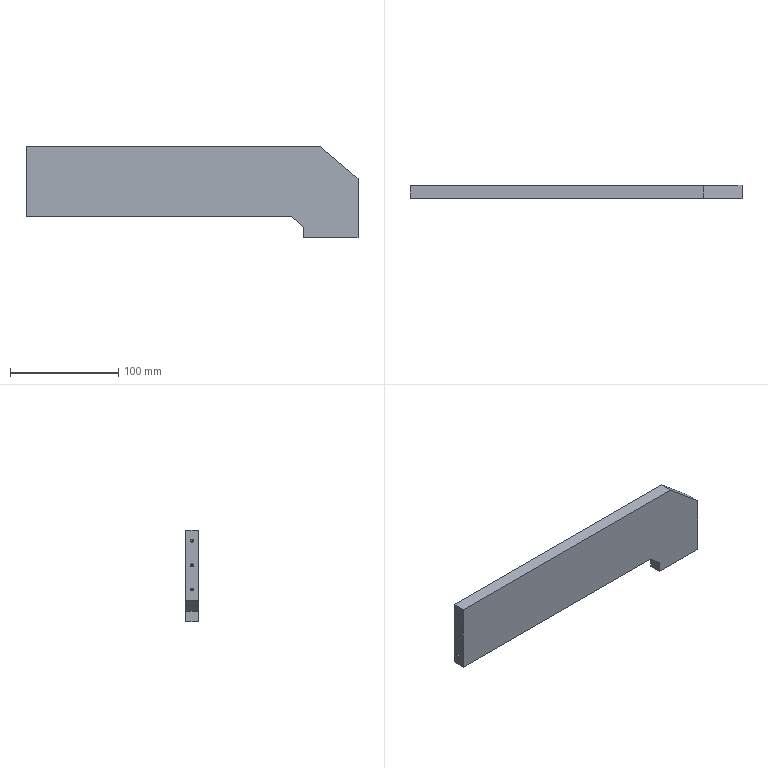Component | SolidWorks | RobotArmCrossPlate1-1 | 1 solid | 34 faces | box 307 x 12 x 85 mm | volume 244874 mm3 | cylinder 12 | cone 12 | plane 10 | commonest cylinder face diameters 4.2 x6 2.5 x6
build123d program:
from build123d import *

# Parameters (mm, degrees)
SKETCH1_W                 = 65
SKETCH1_H                 = 307
BOSS_EXTRUDE1_DEPTH       = 12
SKETCH2_W                 = 85
SKETCH2_H                 = 50
BOSS_EXTRUDE2_DEPTH       = 12
CHAMFER2_SIZE             = 30
CHAMFER2_SIZE2            = 35.753
CHAMFER3_SIZE             = 10
CHAMFER3_SIZE2            = 11.918
M3X0_5_TAPPED_HOLE1_D     = 2.5
M3X0_5_TAPPED_HOLE1_DEPTH = 15
M3X0_5_TAPPED_HOLE1_TIP   = 0.7511
M5X0_8_TAPPED_HOLE1_D     = 4.2
M5X0_8_TAPPED_HOLE1_DEPTH = 15
M5X0_8_TAPPED_HOLE1_TIP   = 1.262


with BuildPart() as part:
    # Sketch1 → Boss-Extrude1 (new body)
    with BuildSketch(Plane.XY):
        Rectangle(SKETCH1_W, SKETCH1_H)
    extrude(amount=BOSS_EXTRUDE1_DEPTH)

    # Sketch2 → Boss-Extrude2 (add)
    with BuildSketch(Plane.XY.offset(12)):
        with Locations((10, 128.5)):
            Rectangle(SKETCH2_W, SKETCH2_H)
    extrude(amount=-BOSS_EXTRUDE2_DEPTH)

    # Chamfer2
    chamfer2_edges = [part.edges().sort_by_distance(p)[0] for p in [
        (-32.5, 153.5, 6),
    ]]
    chamfer2_side = [part.faces().sort_by_distance(p)[0] for p in [
        (10, 153.5, 6),
    ]]
    chamfer(chamfer2_edges, length=CHAMFER2_SIZE, length2=CHAMFER2_SIZE2, reference=chamfer2_side[0])

    # Chamfer3
    chamfer3_edges = [part.edges().sort_by_distance(p)[0] for p in [
        (32.5, 103.5, 6),
    ]]
    chamfer3_side = [part.faces().sort_by_distance(p)[0] for p in [
        (42.5, 103.5, 6),
    ]]
    chamfer(chamfer3_edges, length=CHAMFER3_SIZE, length2=CHAMFER3_SIZE2, reference=chamfer3_side[0])

    # M3x0.5 Tapped Hole1
    with Locations(Plane(origin=(0, -153.5, 0), x_dir=(-1, 0, 0), z_dir=(0, -1, 0))):
        with Locations((22.5, -6), (0, -6), (-22.5, -6)):
            Hole(M3X0_5_TAPPED_HOLE1_D / 2, depth=M3X0_5_TAPPED_HOLE1_DEPTH)
            with Locations((0, 0, -(M3X0_5_TAPPED_HOLE1_DEPTH + M3X0_5_TAPPED_HOLE1_TIP / 2))):  # 118° drill point
                Cone(0, M3X0_5_TAPPED_HOLE1_D / 2, M3X0_5_TAPPED_HOLE1_TIP, mode=Mode.SUBTRACT)

    # M5x0.8 Tapped Hole1
    with Locations(Plane(origin=(52.5, 0, 0), x_dir=(0, 0, -1), z_dir=(1, 0, 0))):
        with Locations((-6, 148.5), (-6, 128.5), (-6.289, 108.5)):
            Hole(M5X0_8_TAPPED_HOLE1_D / 2, depth=M5X0_8_TAPPED_HOLE1_DEPTH)
            with Locations((0, 0, -(M5X0_8_TAPPED_HOLE1_DEPTH + M5X0_8_TAPPED_HOLE1_TIP / 2))):  # 118° drill point
                Cone(0, M5X0_8_TAPPED_HOLE1_D / 2, M5X0_8_TAPPED_HOLE1_TIP, mode=Mode.SUBTRACT)


solid = part.part

# Placed as in the assembly
solid = solid.moved(Location((-174.022, 67.945, 113.051), (90, 0, -90)))
STEP:
#1=COLOUR_RGB('',0.7922,0.8196,0.9333);
#2=FILL_AREA_STYLE_COLOUR('',#1);
#3=FILL_AREA_STYLE('',(#2));
#4=SURFACE_STYLE_FILL_AREA(#3);
#5=SURFACE_SIDE_STYLE('',(#4));
#6=SURFACE_STYLE_USAGE(.BOTH.,#5);
#7=PRESENTATION_STYLE_ASSIGNMENT((#6));
#8=CARTESIAN_POINT('',(-1.005,2.356,2.974));
#9=VERTEX_POINT('',#8);
#10=CARTESIAN_POINT('',(-1.005,2.521,2.974));
#11=VERTEX_POINT('',#10);
#12=CARTESIAN_POINT('',(-1.005,2.439,2.974));
#13=DIRECTION('',(-0.,0.,-1.));
#14=DIRECTION('',(0.,1.,0.));
#15=AXIS2_PLACEMENT_3D('',#12,#13,#14);
#16=CIRCLE('',#15,0.08268);
#17=EDGE_CURVE('',#9,#11,#16,.T.);
#18=ORIENTED_EDGE('',*,*,#17,.F.);
#19=CARTESIAN_POINT('',(-1.005,2.356,2.384));
#20=VERTEX_POINT('',#19);
#21=CARTESIAN_POINT('',(-1.005,2.356,2.384));
#22=DIRECTION('',(-0.,0.,-1.));
#23=VECTOR('',#22,39.37);
#24=LINE('',#21,#23);
#25=EDGE_CURVE('',#9,#20,#24,.T.);
#26=ORIENTED_EDGE('',*,*,#25,.T.);
#27=CARTESIAN_POINT('',(-1.005,2.521,2.384));
#28=VERTEX_POINT('',#27);
#29=CARTESIAN_POINT('',(-1.005,2.439,2.384));
#30=DIRECTION('',(-0.,0.,-1.));
#31=DIRECTION('',(0.,1.,0.));
#32=AXIS2_PLACEMENT_3D('',#29,#30,#31);
#33=CIRCLE('',#32,0.08268);
#34=EDGE_CURVE('',#20,#28,#33,.T.);
#35=ORIENTED_EDGE('',*,*,#34,.T.);
#36=CARTESIAN_POINT('',(-1.005,2.521,2.384));
#37=DIRECTION('',(-0.,0.,-1.));
#38=VECTOR('',#37,39.37);
#39=LINE('',#36,#38);
#40=EDGE_CURVE('',#11,#28,#39,.T.);
#41=ORIENTED_EDGE('',*,*,#40,.F.);
#42=EDGE_LOOP('',(#18,#26,#35,#41));
#43=FACE_OUTER_BOUND('',#42,.T.);
#44=CARTESIAN_POINT('',(-1.005,2.439,2.384));
#45=DIRECTION('',(-0.,0.,-1.));
#46=DIRECTION('',(0.,1.,0.));
#47=AXIS2_PLACEMENT_3D('',#44,#45,#46);
#48=CYLINDRICAL_SURFACE('',#47,0.08268);
#49=ADVANCED_FACE('',(#43),#48,.F.);
#50=CARTESIAN_POINT('',(-1.005,2.439,3.024));
#51=VERTEX_POINT('',#50);
#52=CARTESIAN_POINT('',(-1.005,2.521,2.974));
#53=DIRECTION('',(-0.,0.8572,-0.515));
#54=VECTOR('',#53,39.37);
#55=LINE('',#52,#54);
#56=EDGE_CURVE('',#51,#11,#55,.T.);
#57=ORIENTED_EDGE('',*,*,#56,.F.);
#58=CARTESIAN_POINT('',(-1.005,2.356,2.974));
#59=DIRECTION('',(0.,-0.8572,-0.515));
#60=VECTOR('',#59,39.37);
#61=LINE('',#58,#60);
#62=EDGE_CURVE('',#51,#9,#61,.T.);
#63=ORIENTED_EDGE('',*,*,#62,.T.);
#64=ORIENTED_EDGE('',*,*,#17,.T.);
#65=EDGE_LOOP('',(#57,#63,#64));
#66=FACE_OUTER_BOUND('',#65,.T.);
#67=CARTESIAN_POINT('',(-1.005,2.439,2.974));
#68=DIRECTION('',(-0.,0.,-1.));
#69=DIRECTION('',(0.,1.,0.));
#70=AXIS2_PLACEMENT_3D('',#67,#68,#69);
#71=CONICAL_SURFACE('',#70,0.08268,1.03);
#72=ADVANCED_FACE('',(#66),#71,.F.);
#73=CARTESIAN_POINT('',(-1.792,2.356,2.974));
#74=VERTEX_POINT('',#73);
#75=CARTESIAN_POINT('',(-1.792,2.521,2.974));
#76=VERTEX_POINT('',#75);
#77=CARTESIAN_POINT('',(-1.792,2.439,2.974));
#78=DIRECTION('',(-0.,0.,-1.));
#79=DIRECTION('',(0.,1.,0.));
#80=AXIS2_PLACEMENT_3D('',#77,#78,#79);
#81=CIRCLE('',#80,0.08268);
#82=EDGE_CURVE('',#74,#76,#81,.T.);
#83=ORIENTED_EDGE('',*,*,#82,.F.);
#84=CARTESIAN_POINT('',(-1.792,2.356,2.384));
#85=VERTEX_POINT('',#84);
#86=CARTESIAN_POINT('',(-1.792,2.356,2.384));
#87=DIRECTION('',(-0.,0.,-1.));
#88=VECTOR('',#87,39.37);
#89=LINE('',#86,#88);
#90=EDGE_CURVE('',#74,#85,#89,.T.);
#91=ORIENTED_EDGE('',*,*,#90,.T.);
#92=CARTESIAN_POINT('',(-1.792,2.521,2.384));
#93=VERTEX_POINT('',#92);
#94=CARTESIAN_POINT('',(-1.792,2.439,2.384));
#95=DIRECTION('',(-0.,0.,-1.));
#96=DIRECTION('',(0.,1.,0.));
#97=AXIS2_PLACEMENT_3D('',#94,#95,#96);
#98=CIRCLE('',#97,0.08268);
#99=EDGE_CURVE('',#85,#93,#98,.T.);
#100=ORIENTED_EDGE('',*,*,#99,.T.);
#101=CARTESIAN_POINT('',(-1.792,2.521,2.384));
#102=DIRECTION('',(-0.,0.,-1.));
#103=VECTOR('',#102,39.37);
#104=LINE('',#101,#103);
#105=EDGE_CURVE('',#76,#93,#104,.T.);
#106=ORIENTED_EDGE('',*,*,#105,.F.);
#107=EDGE_LOOP('',(#83,#91,#100,#106));
#108=FACE_OUTER_BOUND('',#107,.T.);
#109=CARTESIAN_POINT('',(-1.792,2.439,2.384));
#110=DIRECTION('',(-0.,0.,-1.));
#111=DIRECTION('',(0.,1.,0.));
#112=AXIS2_PLACEMENT_3D('',#109,#110,#111);
#113=CYLINDRICAL_SURFACE('',#112,0.08268);
#114=ADVANCED_FACE('',(#108),#113,.F.);
#115=CARTESIAN_POINT('',(-1.792,2.439,3.024));
#116=VERTEX_POINT('',#115);
#117=CARTESIAN_POINT('',(-1.792,2.521,2.974));
#118=DIRECTION('',(-0.,0.8572,-0.515));
#119=VECTOR('',#118,39.37);
#120=LINE('',#117,#119);
#121=EDGE_CURVE('',#116,#76,#120,.T.);
#122=ORIENTED_EDGE('',*,*,#121,.F.);
#123=CARTESIAN_POINT('',(-1.792,2.356,2.974));
#124=DIRECTION('',(0.,-0.8572,-0.515));
#125=VECTOR('',#124,39.37);
#126=LINE('',#123,#125);
#127=EDGE_CURVE('',#116,#74,#126,.T.);
#128=ORIENTED_EDGE('',*,*,#127,.T.);
#129=ORIENTED_EDGE('',*,*,#82,.T.);
#130=EDGE_LOOP('',(#122,#128,#129));
#131=FACE_OUTER_BOUND('',#130,.T.);
#132=CARTESIAN_POINT('',(-1.792,2.439,2.974));
#133=DIRECTION('',(-0.,0.,-1.));
#134=DIRECTION('',(0.,1.,0.));
#135=AXIS2_PLACEMENT_3D('',#132,#133,#134);
#136=CONICAL_SURFACE('',#135,0.08268,1.03);
#137=ADVANCED_FACE('',(#131),#136,.F.);
#138=CARTESIAN_POINT('',(-2.58,2.345,2.974));
#139=VERTEX_POINT('',#138);
#140=CARTESIAN_POINT('',(-2.58,2.51,2.974));
#141=VERTEX_POINT('',#140);
#142=CARTESIAN_POINT('',(-2.58,2.427,2.974));
#143=DIRECTION('',(-0.,0.,-1.));
#144=DIRECTION('',(0.,1.,0.));
#145=AXIS2_PLACEMENT_3D('',#142,#143,#144);
#146=CIRCLE('',#145,0.08268);
#147=EDGE_CURVE('',#139,#141,#146,.T.);
#148=ORIENTED_EDGE('',*,*,#147,.F.);
#149=CARTESIAN_POINT('',(-2.58,2.345,2.384));
#150=VERTEX_POINT('',#149);
#151=CARTESIAN_POINT('',(-2.58,2.345,2.384));
#152=DIRECTION('',(-0.,0.,-1.));
#153=VECTOR('',#152,39.37);
#154=LINE('',#151,#153);
#155=EDGE_CURVE('',#139,#150,#154,.T.);
#156=ORIENTED_EDGE('',*,*,#155,.T.);
#157=CARTESIAN_POINT('',(-2.58,2.51,2.384));
#158=VERTEX_POINT('',#157);
#159=CARTESIAN_POINT('',(-2.58,2.427,2.384));
#160=DIRECTION('',(-0.,0.,-1.));
#161=DIRECTION('',(0.,1.,0.));
#162=AXIS2_PLACEMENT_3D('',#159,#160,#161);
#163=CIRCLE('',#162,0.08268);
#164=EDGE_CURVE('',#150,#158,#163,.T.);
#165=ORIENTED_EDGE('',*,*,#164,.T.);
#166=CARTESIAN_POINT('',(-2.58,2.51,2.384));
#167=DIRECTION('',(-0.,0.,-1.));
#168=VECTOR('',#167,39.37);
#169=LINE('',#166,#168);
#170=EDGE_CURVE('',#141,#158,#169,.T.);
#171=ORIENTED_EDGE('',*,*,#170,.F.);
#172=EDGE_LOOP('',(#148,#156,#165,#171));
#173=FACE_OUTER_BOUND('',#172,.T.);
#174=CARTESIAN_POINT('',(-2.58,2.427,2.384));
#175=DIRECTION('',(-0.,0.,-1.));
#176=DIRECTION('',(0.,1.,0.));
#177=AXIS2_PLACEMENT_3D('',#174,#175,#176);
#178=CYLINDRICAL_SURFACE('',#177,0.08268);
#179=ADVANCED_FACE('',(#173),#178,.F.);
#180=CARTESIAN_POINT('',(-2.58,2.427,3.024));
#181=VERTEX_POINT('',#180);
#182=CARTESIAN_POINT('',(-2.58,2.51,2.974));
#183=DIRECTION('',(-0.,0.8572,-0.515));
#184=VECTOR('',#183,39.37);
#185=LINE('',#182,#184);
#186=EDGE_CURVE('',#181,#141,#185,.T.);
#187=ORIENTED_EDGE('',*,*,#186,.F.);
#188=CARTESIAN_POINT('',(-2.58,2.345,2.974));
#189=DIRECTION('',(0.,-0.8572,-0.515));
#190=VECTOR('',#189,39.37);
#191=LINE('',#188,#190);
#192=EDGE_CURVE('',#181,#139,#191,.T.);
#193=ORIENTED_EDGE('',*,*,#192,.T.);
#194=ORIENTED_EDGE('',*,*,#147,.T.);
#195=EDGE_LOOP('',(#187,#193,#194));
#196=FACE_OUTER_BOUND('',#195,.T.);
#197=CARTESIAN_POINT('',(-2.58,2.427,2.974));
#198=DIRECTION('',(-0.,0.,-1.));
#199=DIRECTION('',(0.,1.,0.));
#200=AXIS2_PLACEMENT_3D('',#197,#198,#199);
#201=CONICAL_SURFACE('',#200,0.08268,1.03);
#202=ADVANCED_FACE('',(#196),#201,.F.);
#203=CARTESIAN_POINT('',(-12.304,2.39,5.337));
#204=VERTEX_POINT('',#203);
#205=CARTESIAN_POINT('',(-12.304,2.488,5.337));
#206=VERTEX_POINT('',#205);
#207=CARTESIAN_POINT('',(-12.304,2.439,5.337));
#208=DIRECTION('',(-1.,0.,0.));
#209=DIRECTION('',(0.,1.,0.));
#210=AXIS2_PLACEMENT_3D('',#207,#208,#209);
#211=CIRCLE('',#210,0.04921);
#212=EDGE_CURVE('',#204,#206,#211,.T.);
#213=ORIENTED_EDGE('',*,*,#212,.F.);
#214=CARTESIAN_POINT('',(-12.895,2.39,5.337));
#215=VERTEX_POINT('',#214);
#216=CARTESIAN_POINT('',(-12.895,2.39,5.337));
#217=DIRECTION('',(-1.,0.,0.));
#218=VECTOR('',#217,39.37);
#219=LINE('',#216,#218);
#220=EDGE_CURVE('',#204,#215,#219,.T.);
#221=ORIENTED_EDGE('',*,*,#220,.T.);
#222=CARTESIAN_POINT('',(-12.895,2.488,5.337));
#223=VERTEX_POINT('',#222);
#224=CARTESIAN_POINT('',(-12.895,2.439,5.337));
#225=DIRECTION('',(-1.,0.,0.));
#226=DIRECTION('',(0.,1.,0.));
#227=AXIS2_PLACEMENT_3D('',#224,#225,#226);
#228=CIRCLE('',#227,0.04921);
#229=EDGE_CURVE('',#215,#223,#228,.T.);
#230=ORIENTED_EDGE('',*,*,#229,.T.);
#231=CARTESIAN_POINT('',(-12.895,2.488,5.337));
#232=DIRECTION('',(-1.,0.,0.));
#233=VECTOR('',#232,39.37);
#234=LINE('',#231,#233);
#235=EDGE_CURVE('',#206,#223,#234,.T.);
#236=ORIENTED_EDGE('',*,*,#235,.F.);
#237=EDGE_LOOP('',(#213,#221,#230,#236));
#238=FACE_OUTER_BOUND('',#237,.T.);
#239=CARTESIAN_POINT('',(-12.895,2.439,5.337));
#240=DIRECTION('',(-1.,0.,0.));
#241=DIRECTION('',(0.,1.,0.));
#242=AXIS2_PLACEMENT_3D('',#239,#240,#241);
#243=CYLINDRICAL_SURFACE('',#242,0.04921);
#244=ADVANCED_FACE('',(#238),#243,.F.);
#245=CARTESIAN_POINT('',(-12.274,2.439,5.337));
#246=VERTEX_POINT('',#245);
#247=CARTESIAN_POINT('',(-12.304,2.488,5.337));
#248=DIRECTION('',(-0.515,0.8572,0.));
#249=VECTOR('',#248,39.37);
#250=LINE('',#247,#249);
#251=EDGE_CURVE('',#246,#206,#250,.T.);
#252=ORIENTED_EDGE('',*,*,#251,.F.);
#253=CARTESIAN_POINT('',(-12.304,2.39,5.337));
#254=DIRECTION('',(-0.515,-0.8572,-0.));
#255=VECTOR('',#254,39.37);
#256=LINE('',#253,#255);
#257=EDGE_CURVE('',#246,#204,#256,.T.);
#258=ORIENTED_EDGE('',*,*,#257,.T.);
#259=ORIENTED_EDGE('',*,*,#212,.T.);
#260=EDGE_LOOP('',(#252,#258,#259));
#261=FACE_OUTER_BOUND('',#260,.T.);
#262=CARTESIAN_POINT('',(-12.304,2.439,5.337));
#263=DIRECTION('',(-1.,0.,0.));
#264=DIRECTION('',(0.,1.,0.));
#265=AXIS2_PLACEMENT_3D('',#262,#263,#264);
#266=CONICAL_SURFACE('',#265,0.04921,1.03);
#267=ADVANCED_FACE('',(#261),#266,.F.);
#268=CARTESIAN_POINT('',(-12.304,2.39,4.451));
#269=VERTEX_POINT('',#268);
#270=CARTESIAN_POINT('',(-12.304,2.488,4.451));
#271=VERTEX_POINT('',#270);
#272=CARTESIAN_POINT('',(-12.304,2.439,4.451));
#273=DIRECTION('',(-1.,0.,0.));
#274=DIRECTION('',(0.,1.,0.));
#275=AXIS2_PLACEMENT_3D('',#272,#273,#274);
#276=CIRCLE('',#275,0.04921);
#277=EDGE_CURVE('',#269,#271,#276,.T.);
#278=ORIENTED_EDGE('',*,*,#277,.F.);
#279=CARTESIAN_POINT('',(-12.895,2.39,4.451));
#280=VERTEX_POINT('',#279);
#281=CARTESIAN_POINT('',(-12.895,2.39,4.451));
#282=DIRECTION('',(-1.,0.,0.));
#283=VECTOR('',#282,39.37);
#284=LINE('',#281,#283);
#285=EDGE_CURVE('',#269,#280,#284,.T.);
#286=ORIENTED_EDGE('',*,*,#285,.T.);
#287=CARTESIAN_POINT('',(-12.895,2.488,4.451));
#288=VERTEX_POINT('',#287);
#289=CARTESIAN_POINT('',(-12.895,2.439,4.451));
#290=DIRECTION('',(-1.,0.,0.));
#291=DIRECTION('',(0.,1.,0.));
#292=AXIS2_PLACEMENT_3D('',#289,#290,#291);
#293=CIRCLE('',#292,0.04921);
#294=EDGE_CURVE('',#280,#288,#293,.T.);
#295=ORIENTED_EDGE('',*,*,#294,.T.);
#296=CARTESIAN_POINT('',(-12.895,2.488,4.451));
#297=DIRECTION('',(-1.,0.,0.));
#298=VECTOR('',#297,39.37);
#299=LINE('',#296,#298);
#300=EDGE_CURVE('',#271,#288,#299,.T.);
#301=ORIENTED_EDGE('',*,*,#300,.F.);
#302=EDGE_LOOP('',(#278,#286,#295,#301));
#303=FACE_OUTER_BOUND('',#302,.T.);
#304=CARTESIAN_POINT('',(-12.895,2.439,4.451));
#305=DIRECTION('',(-1.,0.,0.));
#306=DIRECTION('',(0.,1.,0.));
#307=AXIS2_PLACEMENT_3D('',#304,#305,#306);
#308=CYLINDRICAL_SURFACE('',#307,0.04921);
#309=ADVANCED_FACE('',(#303),#308,.F.);
#310=CARTESIAN_POINT('',(-12.274,2.439,4.451));
#311=VERTEX_POINT('',#310);
#312=CARTESIAN_POINT('',(-12.304,2.488,4.451));
#313=DIRECTION('',(-0.515,0.8572,0.));
#314=VECTOR('',#313,39.37);
#315=LINE('',#312,#314);
#316=EDGE_CURVE('',#311,#271,#315,.T.);
#317=ORIENTED_EDGE('',*,*,#316,.F.);
#318=CARTESIAN_POINT('',(-12.304,2.39,4.451));
#319=DIRECTION('',(-0.515,-0.8572,-0.));
#320=VECTOR('',#319,39.37);
#321=LINE('',#318,#320);
#322=EDGE_CURVE('',#311,#269,#321,.T.);
#323=ORIENTED_EDGE('',*,*,#322,.T.);
#324=ORIENTED_EDGE('',*,*,#277,.T.);
#325=EDGE_LOOP('',(#317,#323,#324));
#326=FACE_OUTER_BOUND('',#325,.T.);
#327=CARTESIAN_POINT('',(-12.304,2.439,4.451));
#328=DIRECTION('',(-1.,0.,0.));
#329=DIRECTION('',(0.,1.,0.));
#330=AXIS2_PLACEMENT_3D('',#327,#328,#329);
#331=CONICAL_SURFACE('',#330,0.04921,1.03);
#332=ADVANCED_FACE('',(#326),#331,.F.);
#333=CARTESIAN_POINT('',(-12.304,2.39,3.565));
#334=VERTEX_POINT('',#333);
#335=CARTESIAN_POINT('',(-12.304,2.488,3.565));
#336=VERTEX_POINT('',#335);
#337=CARTESIAN_POINT('',(-12.304,2.439,3.565));
#338=DIRECTION('',(-1.,0.,0.));
#339=DIRECTION('',(0.,1.,0.));
#340=AXIS2_PLACEMENT_3D('',#337,#338,#339);
#341=CIRCLE('',#340,0.04921);
#342=EDGE_CURVE('',#334,#336,#341,.T.);
#343=ORIENTED_EDGE('',*,*,#342,.F.);
#344=CARTESIAN_POINT('',(-12.895,2.39,3.565));
#345=VERTEX_POINT('',#344);
#346=CARTESIAN_POINT('',(-12.895,2.39,3.565));
#347=DIRECTION('',(-1.,0.,0.));
#348=VECTOR('',#347,39.37);
#349=LINE('',#346,#348);
#350=EDGE_CURVE('',#334,#345,#349,.T.);
#351=ORIENTED_EDGE('',*,*,#350,.T.);
#352=CARTESIAN_POINT('',(-12.895,2.488,3.565));
#353=VERTEX_POINT('',#352);
#354=CARTESIAN_POINT('',(-12.895,2.439,3.565));
#355=DIRECTION('',(-1.,0.,0.));
#356=DIRECTION('',(0.,1.,0.));
#357=AXIS2_PLACEMENT_3D('',#354,#355,#356);
#358=CIRCLE('',#357,0.04921);
#359=EDGE_CURVE('',#345,#353,#358,.T.);
#360=ORIENTED_EDGE('',*,*,#359,.T.);
#361=CARTESIAN_POINT('',(-12.895,2.488,3.565));
#362=DIRECTION('',(-1.,0.,0.));
#363=VECTOR('',#362,39.37);
#364=LINE('',#361,#363);
#365=EDGE_CURVE('',#336,#353,#364,.T.);
#366=ORIENTED_EDGE('',*,*,#365,.F.);
#367=EDGE_LOOP('',(#343,#351,#360,#366));
#368=FACE_OUTER_BOUND('',#367,.T.);
#369=CARTESIAN_POINT('',(-12.895,2.439,3.565));
#370=DIRECTION('',(-1.,0.,0.));
#371=DIRECTION('',(0.,1.,0.));
#372=AXIS2_PLACEMENT_3D('',#369,#370,#371);
#373=CYLINDRICAL_SURFACE('',#372,0.04921);
#374=ADVANCED_FACE('',(#368),#373,.F.);
#375=CARTESIAN_POINT('',(-12.274,2.439,3.565));
#376=VERTEX_POINT('',#375);
#377=CARTESIAN_POINT('',(-12.304,2.488,3.565));
#378=DIRECTION('',(-0.515,0.8572,0.));
#379=VECTOR('',#378,39.37);
#380=LINE('',#377,#379);
#381=EDGE_CURVE('',#376,#336,#380,.T.);
#382=ORIENTED_EDGE('',*,*,#381,.F.);
#383=CARTESIAN_POINT('',(-12.304,2.39,3.565));
#384=DIRECTION('',(-0.515,-0.8572,-0.));
#385=VECTOR('',#384,39.37);
#386=LINE('',#383,#385);
#387=EDGE_CURVE('',#376,#334,#386,.T.);
#388=ORIENTED_EDGE('',*,*,#387,.T.);
#389=ORIENTED_EDGE('',*,*,#342,.T.);
#390=EDGE_LOOP('',(#382,#388,#389));
#391=FACE_OUTER_BOUND('',#390,.T.);
#392=CARTESIAN_POINT('',(-12.304,2.439,3.565));
#393=DIRECTION('',(-1.,0.,0.));
#394=DIRECTION('',(0.,1.,0.));
#395=AXIS2_PLACEMENT_3D('',#392,#393,#394);
#396=CONICAL_SURFACE('',#395,0.04921,1.03);
#397=ADVANCED_FACE('',(#391),#396,.F.);
#398=CARTESIAN_POINT('',(-12.895,2.675,3.171));
#399=VERTEX_POINT('',#398);
#400=CARTESIAN_POINT('',(-3.246,2.675,3.171));
#401=VERTEX_POINT('',#400);
#402=CARTESIAN_POINT('',(-0.808,2.675,3.171));
#403=DIRECTION('',(1.,-0.,0.));
#404=VECTOR('',#403,39.37);
#405=LINE('',#402,#404);
#406=EDGE_CURVE('',#399,#401,#405,.T.);
#407=ORIENTED_EDGE('',*,*,#406,.T.);
#408=CARTESIAN_POINT('',(-3.246,2.203,3.171));
#409=VERTEX_POINT('',#408);
#410=CARTESIAN_POINT('',(-3.246,2.203,3.171));
#411=DIRECTION('',(0.,-1.,-0.));
#412=VECTOR('',#411,39.37);
#413=LINE('',#410,#412);
#414=EDGE_CURVE('',#401,#409,#413,.T.);
#415=ORIENTED_EDGE('',*,*,#414,.T.);
#416=CARTESIAN_POINT('',(-12.895,2.203,3.171));
#417=VERTEX_POINT('',#416);
#418=CARTESIAN_POINT('',(-0.808,2.203,3.171));
#419=DIRECTION('',(1.,-0.,0.));
#420=VECTOR('',#419,39.37);
#421=LINE('',#418,#420);
#422=EDGE_CURVE('',#417,#409,#421,.T.);
#423=ORIENTED_EDGE('',*,*,#422,.F.);
#424=CARTESIAN_POINT('',(-12.895,2.203,3.171));
#425=DIRECTION('',(-0.,1.,0.));
#426=VECTOR('',#425,39.37);
#427=LINE('',#424,#426);
#428=EDGE_CURVE('',#417,#399,#427,.T.);
#429=ORIENTED_EDGE('',*,*,#428,.T.);
#430=EDGE_LOOP('',(#407,#415,#423,#429));
#431=FACE_OUTER_BOUND('',#430,.T.);
#432=CARTESIAN_POINT('',(-0.808,2.203,3.171));
#433=DIRECTION('',(-0.,-0.,1.));
#434=DIRECTION('',(-1.,0.,-0.));
#435=AXIS2_PLACEMENT_3D('',#432,#433,#434);
#436=PLANE('',#435);
#437=ADVANCED_FACE('',(#431),#436,.F.);
#438=CARTESIAN_POINT('',(-0.808,2.675,2.384));
#439=VERTEX_POINT('',#438);
#440=CARTESIAN_POINT('',(-0.808,2.675,4.549));
#441=VERTEX_POINT('',#440);
#442=CARTESIAN_POINT('',(-0.808,2.675,5.73));
#443=DIRECTION('',(0.,-0.,1.));
#444=VECTOR('',#443,39.37);
#445=LINE('',#442,#444);
#446=EDGE_CURVE('',#439,#441,#445,.T.);
#447=ORIENTED_EDGE('',*,*,#446,.T.);
#448=CARTESIAN_POINT('',(-0.808,2.203,4.549));
#449=VERTEX_POINT('',#448);
#450=CARTESIAN_POINT('',(-0.808,2.203,4.549));
#451=DIRECTION('',(0.,-1.,-0.));
#452=VECTOR('',#451,39.37);
#453=LINE('',#450,#452);
#454=EDGE_CURVE('',#441,#449,#453,.T.);
#455=ORIENTED_EDGE('',*,*,#454,.T.);
#456=CARTESIAN_POINT('',(-0.808,2.203,2.384));
#457=VERTEX_POINT('',#456);
#458=CARTESIAN_POINT('',(-0.808,2.203,5.73));
#459=DIRECTION('',(0.,-0.,1.));
#460=VECTOR('',#459,39.37);
#461=LINE('',#458,#460);
#462=EDGE_CURVE('',#457,#449,#461,.T.);
#463=ORIENTED_EDGE('',*,*,#462,.F.);
#464=CARTESIAN_POINT('',(-0.808,2.675,2.384));
#465=DIRECTION('',(0.,-1.,-0.));
#466=VECTOR('',#465,39.37);
#467=LINE('',#464,#466);
#468=EDGE_CURVE('',#439,#457,#467,.T.);
#469=ORIENTED_EDGE('',*,*,#468,.F.);
#470=EDGE_LOOP('',(#447,#455,#463,#469));
#471=FACE_OUTER_BOUND('',#470,.T.);
#472=CARTESIAN_POINT('',(-0.808,2.203,5.73));
#473=DIRECTION('',(-1.,-0.,0.));
#474=DIRECTION('',(-0.,1.,0.));
#475=AXIS2_PLACEMENT_3D('',#472,#473,#474);
#476=PLANE('',#475);
#477=ADVANCED_FACE('',(#471),#476,.F.);
#478=CARTESIAN_POINT('',(-2.216,2.203,5.73));
#479=VERTEX_POINT('',#478);
#480=CARTESIAN_POINT('',(-12.895,2.203,5.73));
#481=VERTEX_POINT('',#480);
#482=CARTESIAN_POINT('',(-0.808,2.203,5.73));
#483=DIRECTION('',(-1.,0.,-0.));
#484=VECTOR('',#483,39.37);
#485=LINE('',#482,#484);
#486=EDGE_CURVE('',#479,#481,#485,.T.);
#487=ORIENTED_EDGE('',*,*,#486,.F.);
#488=CARTESIAN_POINT('',(-2.216,2.675,5.73));
#489=VERTEX_POINT('',#488);
#490=CARTESIAN_POINT('',(-2.216,2.203,5.73));
#491=DIRECTION('',(-0.,1.,0.));
#492=VECTOR('',#491,39.37);
#493=LINE('',#490,#492);
#494=EDGE_CURVE('',#479,#489,#493,.T.);
#495=ORIENTED_EDGE('',*,*,#494,.T.);
#496=CARTESIAN_POINT('',(-12.895,2.675,5.73));
#497=VERTEX_POINT('',#496);
#498=CARTESIAN_POINT('',(-0.808,2.675,5.73));
#499=DIRECTION('',(-1.,0.,-0.));
#500=VECTOR('',#499,39.37);
#501=LINE('',#498,#500);
#502=EDGE_CURVE('',#489,#497,#501,.T.);
#503=ORIENTED_EDGE('',*,*,#502,.T.);
#504=CARTESIAN_POINT('',(-12.895,2.203,5.73));
#505=DIRECTION('',(-0.,1.,0.));
#506=VECTOR('',#505,39.37);
#507=LINE('',#504,#506);
#508=EDGE_CURVE('',#481,#497,#507,.T.);
#509=ORIENTED_EDGE('',*,*,#508,.F.);
#510=EDGE_LOOP('',(#487,#495,#503,#509));
#511=FACE_OUTER_BOUND('',#510,.T.);
#512=CARTESIAN_POINT('',(-0.808,2.203,5.73));
#513=DIRECTION('',(0.,0.,-1.));
#514=DIRECTION('',(1.,-0.,0.));
#515=AXIS2_PLACEMENT_3D('',#512,#513,#514);
#516=PLANE('',#515);
#517=ADVANCED_FACE('',(#511),#516,.F.);
#518=CARTESIAN_POINT('',(-12.895,2.439,5.337));
#519=DIRECTION('',(-1.,0.,0.));
#520=DIRECTION('',(0.,1.,0.));
#521=AXIS2_PLACEMENT_3D('',#518,#519,#520);
#522=CIRCLE('',#521,0.04921);
#523=EDGE_CURVE('',#223,#215,#522,.T.);
#524=ORIENTED_EDGE('',*,*,#523,.F.);
#525=ORIENTED_EDGE('',*,*,#229,.F.);
#526=EDGE_LOOP('',(#524,#525));
#527=FACE_BOUND('',#526,.T.);
#528=CARTESIAN_POINT('',(-12.895,2.439,4.451));
#529=DIRECTION('',(-1.,0.,0.));
#530=DIRECTION('',(0.,1.,0.));
#531=AXIS2_PLACEMENT_3D('',#528,#529,#530);
#532=CIRCLE('',#531,0.04921);
#533=EDGE_CURVE('',#288,#280,#532,.T.);
#534=ORIENTED_EDGE('',*,*,#533,.F.);
#535=ORIENTED_EDGE('',*,*,#294,.F.);
#536=EDGE_LOOP('',(#534,#535));
#537=FACE_BOUND('',#536,.T.);
#538=CARTESIAN_POINT('',(-12.895,2.439,3.565));
#539=DIRECTION('',(-1.,0.,0.));
#540=DIRECTION('',(0.,1.,0.));
#541=AXIS2_PLACEMENT_3D('',#538,#539,#540);
#542=CIRCLE('',#541,0.04921);
#543=EDGE_CURVE('',#353,#345,#542,.T.);
#544=ORIENTED_EDGE('',*,*,#543,.F.);
#545=ORIENTED_EDGE('',*,*,#359,.F.);
#546=EDGE_LOOP('',(#544,#545));
#547=FACE_BOUND('',#546,.T.);
#548=CARTESIAN_POINT('',(-12.895,2.675,5.73));
#549=DIRECTION('',(-0.,0.,-1.));
#550=VECTOR('',#549,39.37);
#551=LINE('',#548,#550);
#552=EDGE_CURVE('',#497,#399,#551,.T.);
#553=ORIENTED_EDGE('',*,*,#552,.T.);
#554=ORIENTED_EDGE('',*,*,#428,.F.);
#555=CARTESIAN_POINT('',(-12.895,2.203,5.73));
#556=DIRECTION('',(-0.,0.,-1.));
#557=VECTOR('',#556,39.37);
#558=LINE('',#555,#557);
#559=EDGE_CURVE('',#481,#417,#558,.T.);
#560=ORIENTED_EDGE('',*,*,#559,.F.);
#561=ORIENTED_EDGE('',*,*,#508,.T.);
#562=EDGE_LOOP('',(#553,#554,#560,#561));
#563=FACE_OUTER_BOUND('',#562,.T.);
#564=CARTESIAN_POINT('',(-12.895,2.203,5.73));
#565=DIRECTION('',(1.,0.,-0.));
#566=DIRECTION('',(0.,-1.,-0.));
#567=AXIS2_PLACEMENT_3D('',#564,#565,#566);
#568=PLANE('',#567);
#569=ADVANCED_FACE('',(#527,#537,#547,#563),#568,.F.);
#570=ORIENTED_EDGE('',*,*,#462,.T.);
#571=CARTESIAN_POINT('',(-4.306,2.203,7.484));
#572=DIRECTION('',(-0.766,-0.,0.6428));
#573=VECTOR('',#572,39.37);
#574=LINE('',#571,#573);
#575=EDGE_CURVE('',#449,#479,#574,.T.);
#576=ORIENTED_EDGE('',*,*,#575,.T.);
#577=ORIENTED_EDGE('',*,*,#486,.T.);
#578=ORIENTED_EDGE('',*,*,#559,.T.);
#579=ORIENTED_EDGE('',*,*,#422,.T.);
#580=CARTESIAN_POINT('',(-2.776,2.203,2.778));
#581=VERTEX_POINT('',#580);
#582=CARTESIAN_POINT('',(-3.246,2.203,3.171));
#583=DIRECTION('',(0.766,0.,-0.6428));
#584=VECTOR('',#583,39.37);
#585=LINE('',#582,#584);
#586=EDGE_CURVE('',#409,#581,#585,.T.);
#587=ORIENTED_EDGE('',*,*,#586,.T.);
#588=CARTESIAN_POINT('',(-2.776,2.203,2.384));
#589=VERTEX_POINT('',#588);
#590=CARTESIAN_POINT('',(-2.776,2.203,5.73));
#591=DIRECTION('',(-0.,0.,-1.));
#592=VECTOR('',#591,39.37);
#593=LINE('',#590,#592);
#594=EDGE_CURVE('',#581,#589,#593,.T.);
#595=ORIENTED_EDGE('',*,*,#594,.T.);
#596=CARTESIAN_POINT('',(-0.808,2.203,2.384));
#597=DIRECTION('',(1.,-0.,0.));
#598=VECTOR('',#597,39.37);
#599=LINE('',#596,#598);
#600=EDGE_CURVE('',#589,#457,#599,.T.);
#601=ORIENTED_EDGE('',*,*,#600,.T.);
#602=EDGE_LOOP('',(#570,#576,#577,#578,#579,#587,#595,#601));
#603=FACE_OUTER_BOUND('',#602,.T.);
#604=CARTESIAN_POINT('',(-6.851,2.203,4.451));
#605=DIRECTION('',(0.,-1.,-0.));
#606=DIRECTION('',(-0.,0.,-1.));
#607=AXIS2_PLACEMENT_3D('',#604,#605,#606);
#608=PLANE('',#607);
#609=ADVANCED_FACE('',(#603),#608,.T.);
#610=ORIENTED_EDGE('',*,*,#502,.F.);
#611=CARTESIAN_POINT('',(-2.216,2.675,5.73));
#612=DIRECTION('',(0.766,0.,-0.6428));
#613=VECTOR('',#612,39.37);
#614=LINE('',#611,#613);
#615=EDGE_CURVE('',#489,#441,#614,.T.);
#616=ORIENTED_EDGE('',*,*,#615,.T.);
#617=ORIENTED_EDGE('',*,*,#446,.F.);
#618=CARTESIAN_POINT('',(-2.776,2.675,2.384));
#619=VERTEX_POINT('',#618);
#620=CARTESIAN_POINT('',(-0.808,2.675,2.384));
#621=DIRECTION('',(1.,-0.,0.));
#622=VECTOR('',#621,39.37);
#623=LINE('',#620,#622);
#624=EDGE_CURVE('',#619,#439,#623,.T.);
#625=ORIENTED_EDGE('',*,*,#624,.F.);
#626=CARTESIAN_POINT('',(-2.776,2.675,2.778));
#627=VERTEX_POINT('',#626);
#628=CARTESIAN_POINT('',(-2.776,2.675,5.73));
#629=DIRECTION('',(-0.,0.,-1.));
#630=VECTOR('',#629,39.37);
#631=LINE('',#628,#630);
#632=EDGE_CURVE('',#627,#619,#631,.T.);
#633=ORIENTED_EDGE('',*,*,#632,.F.);
#634=CARTESIAN_POINT('',(-5.992,2.675,5.475));
#635=DIRECTION('',(-0.766,-0.,0.6428));
#636=VECTOR('',#635,39.37);
#637=LINE('',#634,#636);
#638=EDGE_CURVE('',#627,#401,#637,.T.);
#639=ORIENTED_EDGE('',*,*,#638,.T.);
#640=ORIENTED_EDGE('',*,*,#406,.F.);
#641=ORIENTED_EDGE('',*,*,#552,.F.);
#642=EDGE_LOOP('',(#610,#616,#617,#625,#633,#639,#640,#641));
#643=FACE_OUTER_BOUND('',#642,.T.);
#644=CARTESIAN_POINT('',(-6.851,2.675,4.451));
#645=DIRECTION('',(0.,-1.,-0.));
#646=DIRECTION('',(-0.,0.,-1.));
#647=AXIS2_PLACEMENT_3D('',#644,#645,#646);
#648=PLANE('',#647);
#649=ADVANCED_FACE('',(#643),#648,.F.);
#650=ORIENTED_EDGE('',*,*,#594,.F.);
#651=CARTESIAN_POINT('',(-2.776,2.675,2.778));
#652=DIRECTION('',(-0.,1.,0.));
#653=VECTOR('',#652,39.37);
#654=LINE('',#651,#653);
#655=EDGE_CURVE('',#581,#627,#654,.T.);
#656=ORIENTED_EDGE('',*,*,#655,.T.);
#657=ORIENTED_EDGE('',*,*,#632,.T.);
#658=CARTESIAN_POINT('',(-2.776,2.675,2.384));
#659=DIRECTION('',(0.,-1.,-0.));
#660=VECTOR('',#659,39.37);
#661=LINE('',#658,#660);
#662=EDGE_CURVE('',#619,#589,#661,.T.);
#663=ORIENTED_EDGE('',*,*,#662,.T.);
#664=EDGE_LOOP('',(#650,#656,#657,#663));
#665=FACE_OUTER_BOUND('',#664,.T.);
#666=CARTESIAN_POINT('',(-2.776,2.675,5.73));
#667=DIRECTION('',(-1.,-0.,0.));
#668=DIRECTION('',(-0.,1.,0.));
#669=AXIS2_PLACEMENT_3D('',#666,#667,#668);
#670=PLANE('',#669);
#671=ADVANCED_FACE('',(#665),#670,.T.);
#672=CARTESIAN_POINT('',(-1.005,2.439,2.384));
#673=DIRECTION('',(-0.,0.,-1.));
#674=DIRECTION('',(0.,1.,0.));
#675=AXIS2_PLACEMENT_3D('',#672,#673,#674);
#676=CIRCLE('',#675,0.08268);
#677=EDGE_CURVE('',#28,#20,#676,.T.);
#678=ORIENTED_EDGE('',*,*,#677,.F.);
#679=ORIENTED_EDGE('',*,*,#34,.F.);
#680=EDGE_LOOP('',(#678,#679));
#681=FACE_BOUND('',#680,.T.);
#682=CARTESIAN_POINT('',(-1.792,2.439,2.384));
#683=DIRECTION('',(-0.,0.,-1.));
#684=DIRECTION('',(0.,1.,0.));
#685=AXIS2_PLACEMENT_3D('',#682,#683,#684);
#686=CIRCLE('',#685,0.08268);
#687=EDGE_CURVE('',#93,#85,#686,.T.);
#688=ORIENTED_EDGE('',*,*,#687,.F.);
#689=ORIENTED_EDGE('',*,*,#99,.F.);
#690=EDGE_LOOP('',(#688,#689));
#691=FACE_BOUND('',#690,.T.);
#692=CARTESIAN_POINT('',(-2.58,2.427,2.384));
#693=DIRECTION('',(-0.,0.,-1.));
#694=DIRECTION('',(0.,1.,0.));
#695=AXIS2_PLACEMENT_3D('',#692,#693,#694);
#696=CIRCLE('',#695,0.08268);
#697=EDGE_CURVE('',#158,#150,#696,.T.);
#698=ORIENTED_EDGE('',*,*,#697,.F.);
#699=ORIENTED_EDGE('',*,*,#164,.F.);
#700=EDGE_LOOP('',(#698,#699));
#701=FACE_BOUND('',#700,.T.);
#702=ORIENTED_EDGE('',*,*,#600,.F.);
#703=ORIENTED_EDGE('',*,*,#662,.F.);
#704=ORIENTED_EDGE('',*,*,#624,.T.);
#705=ORIENTED_EDGE('',*,*,#468,.T.);
#706=EDGE_LOOP('',(#702,#703,#704,#705));
#707=FACE_OUTER_BOUND('',#706,.T.);
#708=CARTESIAN_POINT('',(-0.808,2.675,2.384));
#709=DIRECTION('',(0.,0.,-1.));
#710=DIRECTION('',(1.,-0.,0.));
#711=AXIS2_PLACEMENT_3D('',#708,#709,#710);
#712=PLANE('',#711);
#713=ADVANCED_FACE('',(#681,#691,#701,#707),#712,.T.);
#714=ORIENTED_EDGE('',*,*,#575,.F.);
#715=ORIENTED_EDGE('',*,*,#454,.F.);
#716=ORIENTED_EDGE('',*,*,#615,.F.);
#717=ORIENTED_EDGE('',*,*,#494,.F.);
#718=EDGE_LOOP('',(#714,#715,#716,#717));
#719=FACE_OUTER_BOUND('',#718,.T.);
#720=CARTESIAN_POINT('',(-2.216,2.203,5.73));
#721=DIRECTION('',(-0.6428,0.,-0.766));
#722=DIRECTION('',(-0.,1.,0.));
#723=AXIS2_PLACEMENT_3D('',#720,#721,#722);
#724=PLANE('',#723);
#725=ADVANCED_FACE('',(#719),#724,.F.);
#726=ORIENTED_EDGE('',*,*,#638,.F.);
#727=ORIENTED_EDGE('',*,*,#655,.F.);
#728=ORIENTED_EDGE('',*,*,#586,.F.);
#729=ORIENTED_EDGE('',*,*,#414,.F.);
#730=EDGE_LOOP('',(#726,#727,#728,#729));
#731=FACE_OUTER_BOUND('',#730,.T.);
#732=CARTESIAN_POINT('',(-3.246,2.203,3.171));
#733=DIRECTION('',(0.6428,-0.,0.766));
#734=DIRECTION('',(0.,-1.,-0.));
#735=AXIS2_PLACEMENT_3D('',#732,#733,#734);
#736=PLANE('',#735);
#737=ADVANCED_FACE('',(#731),#736,.F.);
#738=ORIENTED_EDGE('',*,*,#387,.F.);
#739=ORIENTED_EDGE('',*,*,#381,.T.);
#740=CARTESIAN_POINT('',(-12.304,2.439,3.565));
#741=DIRECTION('',(-1.,0.,0.));
#742=DIRECTION('',(0.,1.,0.));
#743=AXIS2_PLACEMENT_3D('',#740,#741,#742);
#744=CIRCLE('',#743,0.04921);
#745=EDGE_CURVE('',#336,#334,#744,.T.);
#746=ORIENTED_EDGE('',*,*,#745,.T.);
#747=EDGE_LOOP('',(#738,#739,#746));
#748=FACE_OUTER_BOUND('',#747,.T.);
#749=CARTESIAN_POINT('',(-12.304,2.439,3.565));
#750=DIRECTION('',(-1.,0.,0.));
#751=DIRECTION('',(0.,1.,0.));
#752=AXIS2_PLACEMENT_3D('',#749,#750,#751);
#753=CONICAL_SURFACE('',#752,0.04921,1.03);
#754=ADVANCED_FACE('',(#748),#753,.F.);
#755=ORIENTED_EDGE('',*,*,#350,.F.);
#756=ORIENTED_EDGE('',*,*,#745,.F.);
#757=ORIENTED_EDGE('',*,*,#365,.T.);
#758=ORIENTED_EDGE('',*,*,#543,.T.);
#759=EDGE_LOOP('',(#755,#756,#757,#758));
#760=FACE_OUTER_BOUND('',#759,.T.);
#761=CARTESIAN_POINT('',(-12.895,2.439,3.565));
#762=DIRECTION('',(-1.,0.,0.));
#763=DIRECTION('',(0.,1.,0.));
#764=AXIS2_PLACEMENT_3D('',#761,#762,#763);
#765=CYLINDRICAL_SURFACE('',#764,0.04921);
#766=ADVANCED_FACE('',(#760),#765,.F.);
#767=ORIENTED_EDGE('',*,*,#322,.F.);
#768=ORIENTED_EDGE('',*,*,#316,.T.);
#769=CARTESIAN_POINT('',(-12.304,2.439,4.451));
#770=DIRECTION('',(-1.,0.,0.));
#771=DIRECTION('',(0.,1.,0.));
#772=AXIS2_PLACEMENT_3D('',#769,#770,#771);
#773=CIRCLE('',#772,0.04921);
#774=EDGE_CURVE('',#271,#269,#773,.T.);
#775=ORIENTED_EDGE('',*,*,#774,.T.);
#776=EDGE_LOOP('',(#767,#768,#775));
#777=FACE_OUTER_BOUND('',#776,.T.);
#778=CARTESIAN_POINT('',(-12.304,2.439,4.451));
#779=DIRECTION('',(-1.,0.,0.));
#780=DIRECTION('',(0.,1.,0.));
#781=AXIS2_PLACEMENT_3D('',#778,#779,#780);
#782=CONICAL_SURFACE('',#781,0.04921,1.03);
#783=ADVANCED_FACE('',(#777),#782,.F.);
#784=ORIENTED_EDGE('',*,*,#285,.F.);
#785=ORIENTED_EDGE('',*,*,#774,.F.);
#786=ORIENTED_EDGE('',*,*,#300,.T.);
#787=ORIENTED_EDGE('',*,*,#533,.T.);
#788=EDGE_LOOP('',(#784,#785,#786,#787));
#789=FACE_OUTER_BOUND('',#788,.T.);
#790=CARTESIAN_POINT('',(-12.895,2.439,4.451));
#791=DIRECTION('',(-1.,0.,0.));
#792=DIRECTION('',(0.,1.,0.));
#793=AXIS2_PLACEMENT_3D('',#790,#791,#792);
#794=CYLINDRICAL_SURFACE('',#793,0.04921);
#795=ADVANCED_FACE('',(#789),#794,.F.);
#796=ORIENTED_EDGE('',*,*,#257,.F.);
#797=ORIENTED_EDGE('',*,*,#251,.T.);
#798=CARTESIAN_POINT('',(-12.304,2.439,5.337));
#799=DIRECTION('',(-1.,0.,0.));
#800=DIRECTION('',(0.,1.,0.));
#801=AXIS2_PLACEMENT_3D('',#798,#799,#800);
#802=CIRCLE('',#801,0.04921);
#803=EDGE_CURVE('',#206,#204,#802,.T.);
#804=ORIENTED_EDGE('',*,*,#803,.T.);
#805=EDGE_LOOP('',(#796,#797,#804));
#806=FACE_OUTER_BOUND('',#805,.T.);
#807=CARTESIAN_POINT('',(-12.304,2.439,5.337));
#808=DIRECTION('',(-1.,0.,0.));
#809=DIRECTION('',(0.,1.,0.));
#810=AXIS2_PLACEMENT_3D('',#807,#808,#809);
#811=CONICAL_SURFACE('',#810,0.04921,1.03);
#812=ADVANCED_FACE('',(#806),#811,.F.);
#813=ORIENTED_EDGE('',*,*,#220,.F.);
#814=ORIENTED_EDGE('',*,*,#803,.F.);
#815=ORIENTED_EDGE('',*,*,#235,.T.);
#816=ORIENTED_EDGE('',*,*,#523,.T.);
#817=EDGE_LOOP('',(#813,#814,#815,#816));
#818=FACE_OUTER_BOUND('',#817,.T.);
#819=CARTESIAN_POINT('',(-12.895,2.439,5.337));
#820=DIRECTION('',(-1.,0.,0.));
#821=DIRECTION('',(0.,1.,0.));
#822=AXIS2_PLACEMENT_3D('',#819,#820,#821);
#823=CYLINDRICAL_SURFACE('',#822,0.04921);
#824=ADVANCED_FACE('',(#818),#823,.F.);
#825=ORIENTED_EDGE('',*,*,#192,.F.);
#826=ORIENTED_EDGE('',*,*,#186,.T.);
#827=CARTESIAN_POINT('',(-2.58,2.427,2.974));
#828=DIRECTION('',(-0.,0.,-1.));
#829=DIRECTION('',(0.,1.,0.));
#830=AXIS2_PLACEMENT_3D('',#827,#828,#829);
#831=CIRCLE('',#830,0.08268);
#832=EDGE_CURVE('',#141,#139,#831,.T.);
#833=ORIENTED_EDGE('',*,*,#832,.T.);
#834=EDGE_LOOP('',(#825,#826,#833));
#835=FACE_OUTER_BOUND('',#834,.T.);
#836=CARTESIAN_POINT('',(-2.58,2.427,2.974));
#837=DIRECTION('',(-0.,0.,-1.));
#838=DIRECTION('',(0.,1.,0.));
#839=AXIS2_PLACEMENT_3D('',#836,#837,#838);
#840=CONICAL_SURFACE('',#839,0.08268,1.03);
#841=ADVANCED_FACE('',(#835),#840,.F.);
#842=ORIENTED_EDGE('',*,*,#155,.F.);
#843=ORIENTED_EDGE('',*,*,#832,.F.);
#844=ORIENTED_EDGE('',*,*,#170,.T.);
#845=ORIENTED_EDGE('',*,*,#697,.T.);
#846=EDGE_LOOP('',(#842,#843,#844,#845));
#847=FACE_OUTER_BOUND('',#846,.T.);
#848=CARTESIAN_POINT('',(-2.58,2.427,2.384));
#849=DIRECTION('',(-0.,0.,-1.));
#850=DIRECTION('',(0.,1.,0.));
#851=AXIS2_PLACEMENT_3D('',#848,#849,#850);
#852=CYLINDRICAL_SURFACE('',#851,0.08268);
#853=ADVANCED_FACE('',(#847),#852,.F.);
#854=ORIENTED_EDGE('',*,*,#127,.F.);
#855=ORIENTED_EDGE('',*,*,#121,.T.);
#856=CARTESIAN_POINT('',(-1.792,2.439,2.974));
#857=DIRECTION('',(-0.,0.,-1.));
#858=DIRECTION('',(0.,1.,0.));
#859=AXIS2_PLACEMENT_3D('',#856,#857,#858);
#860=CIRCLE('',#859,0.08268);
#861=EDGE_CURVE('',#76,#74,#860,.T.);
#862=ORIENTED_EDGE('',*,*,#861,.T.);
#863=EDGE_LOOP('',(#854,#855,#862));
#864=FACE_OUTER_BOUND('',#863,.T.);
#865=CARTESIAN_POINT('',(-1.792,2.439,2.974));
#866=DIRECTION('',(-0.,0.,-1.));
#867=DIRECTION('',(0.,1.,0.));
#868=AXIS2_PLACEMENT_3D('',#865,#866,#867);
#869=CONICAL_SURFACE('',#868,0.08268,1.03);
#870=ADVANCED_FACE('',(#864),#869,.F.);
#871=ORIENTED_EDGE('',*,*,#90,.F.);
#872=ORIENTED_EDGE('',*,*,#861,.F.);
#873=ORIENTED_EDGE('',*,*,#105,.T.);
#874=ORIENTED_EDGE('',*,*,#687,.T.);
#875=EDGE_LOOP('',(#871,#872,#873,#874));
#876=FACE_OUTER_BOUND('',#875,.T.);
#877=CARTESIAN_POINT('',(-1.792,2.439,2.384));
#878=DIRECTION('',(-0.,0.,-1.));
#879=DIRECTION('',(0.,1.,0.));
#880=AXIS2_PLACEMENT_3D('',#877,#878,#879);
#881=CYLINDRICAL_SURFACE('',#880,0.08268);
#882=ADVANCED_FACE('',(#876),#881,.F.);
#883=ORIENTED_EDGE('',*,*,#62,.F.);
#884=ORIENTED_EDGE('',*,*,#56,.T.);
#885=CARTESIAN_POINT('',(-1.005,2.439,2.974));
#886=DIRECTION('',(-0.,0.,-1.));
#887=DIRECTION('',(0.,1.,0.));
#888=AXIS2_PLACEMENT_3D('',#885,#886,#887);
#889=CIRCLE('',#888,0.08268);
#890=EDGE_CURVE('',#11,#9,#889,.T.);
#891=ORIENTED_EDGE('',*,*,#890,.T.);
#892=EDGE_LOOP('',(#883,#884,#891));
#893=FACE_OUTER_BOUND('',#892,.T.);
#894=CARTESIAN_POINT('',(-1.005,2.439,2.974));
#895=DIRECTION('',(-0.,0.,-1.));
#896=DIRECTION('',(0.,1.,0.));
#897=AXIS2_PLACEMENT_3D('',#894,#895,#896);
#898=CONICAL_SURFACE('',#897,0.08268,1.03);
#899=ADVANCED_FACE('',(#893),#898,.F.);
#900=ORIENTED_EDGE('',*,*,#25,.F.);
#901=ORIENTED_EDGE('',*,*,#890,.F.);
#902=ORIENTED_EDGE('',*,*,#40,.T.);
#903=ORIENTED_EDGE('',*,*,#677,.T.);
#904=EDGE_LOOP('',(#900,#901,#902,#903));
#905=FACE_OUTER_BOUND('',#904,.T.);
#906=CARTESIAN_POINT('',(-1.005,2.439,2.384));
#907=DIRECTION('',(-0.,0.,-1.));
#908=DIRECTION('',(0.,1.,0.));
#909=AXIS2_PLACEMENT_3D('',#906,#907,#908);
#910=CYLINDRICAL_SURFACE('',#909,0.08268);
#911=ADVANCED_FACE('',(#905),#910,.F.);
#912=CLOSED_SHELL('',(#49,#72,#114,#137,#179,#202,#244,#267,#309,#332,#374,#397,#437,#477,#517,#569,#609,#649,#671,#713,#725,#737,#754,#766,#783,#795,#812,#824,#841,#853,#870,#882,#899,#911));
#913=MANIFOLD_SOLID_BREP('',#912);
#914=STYLED_ITEM('',(#7),#913);
#915=PRESENTATION_LAYER_ASSIGNMENT('','',(#914));
#916=(LENGTH_UNIT()NAMED_UNIT(*)SI_UNIT($,.METRE.));
#917=LENGTH_MEASURE_WITH_UNIT(LENGTH_MEASURE(0.0254),#916);
#918=DIMENSIONAL_EXPONENTS(1.,0.,0.,0.,0.,0.,0.);
#919=(CONVERSION_BASED_UNIT('',#917)LENGTH_UNIT()NAMED_UNIT(#918));
#920=UNCERTAINTY_MEASURE_WITH_UNIT(LENGTH_MEASURE(0.00001),#919,'','');
#921=(NAMED_UNIT(*)PLANE_ANGLE_UNIT()SI_UNIT($,.RADIAN.));
#922=(NAMED_UNIT(*)SI_UNIT($,.STERADIAN.)SOLID_ANGLE_UNIT());
#923=(GEOMETRIC_REPRESENTATION_CONTEXT(3)GLOBAL_UNCERTAINTY_ASSIGNED_CONTEXT((#920))GLOBAL_UNIT_ASSIGNED_CONTEXT((#919,#921,#922))REPRESENTATION_CONTEXT('',''));
#924=MECHANICAL_DESIGN_GEOMETRIC_PRESENTATION_REPRESENTATION('',(#914),#923);
#925=CARTESIAN_POINT('',(0.,0.,0.));
#926=DIRECTION('',(0.,0.,1.));
#927=DIRECTION('',(1.,0.,0.));
#928=AXIS2_PLACEMENT_3D('',#925,#926,#927);
#929=(LENGTH_UNIT()NAMED_UNIT(*)SI_UNIT($,.METRE.));
#930=LENGTH_MEASURE_WITH_UNIT(LENGTH_MEASURE(0.0254),#929);
#931=DIMENSIONAL_EXPONENTS(1.,0.,0.,0.,0.,0.,0.);
#932=(CONVERSION_BASED_UNIT('',#930)LENGTH_UNIT()NAMED_UNIT(#931));
#933=UNCERTAINTY_MEASURE_WITH_UNIT(LENGTH_MEASURE(0.00001),#932,'','');
#934=(NAMED_UNIT(*)PLANE_ANGLE_UNIT()SI_UNIT($,.RADIAN.));
#935=(NAMED_UNIT(*)SI_UNIT($,.STERADIAN.)SOLID_ANGLE_UNIT());
#936=(GEOMETRIC_REPRESENTATION_CONTEXT(3)GLOBAL_UNCERTAINTY_ASSIGNED_CONTEXT((#933))GLOBAL_UNIT_ASSIGNED_CONTEXT((#932,#934,#935))REPRESENTATION_CONTEXT('',''));
#937=ADVANCED_BREP_SHAPE_REPRESENTATION('',(#913,#928),#936);